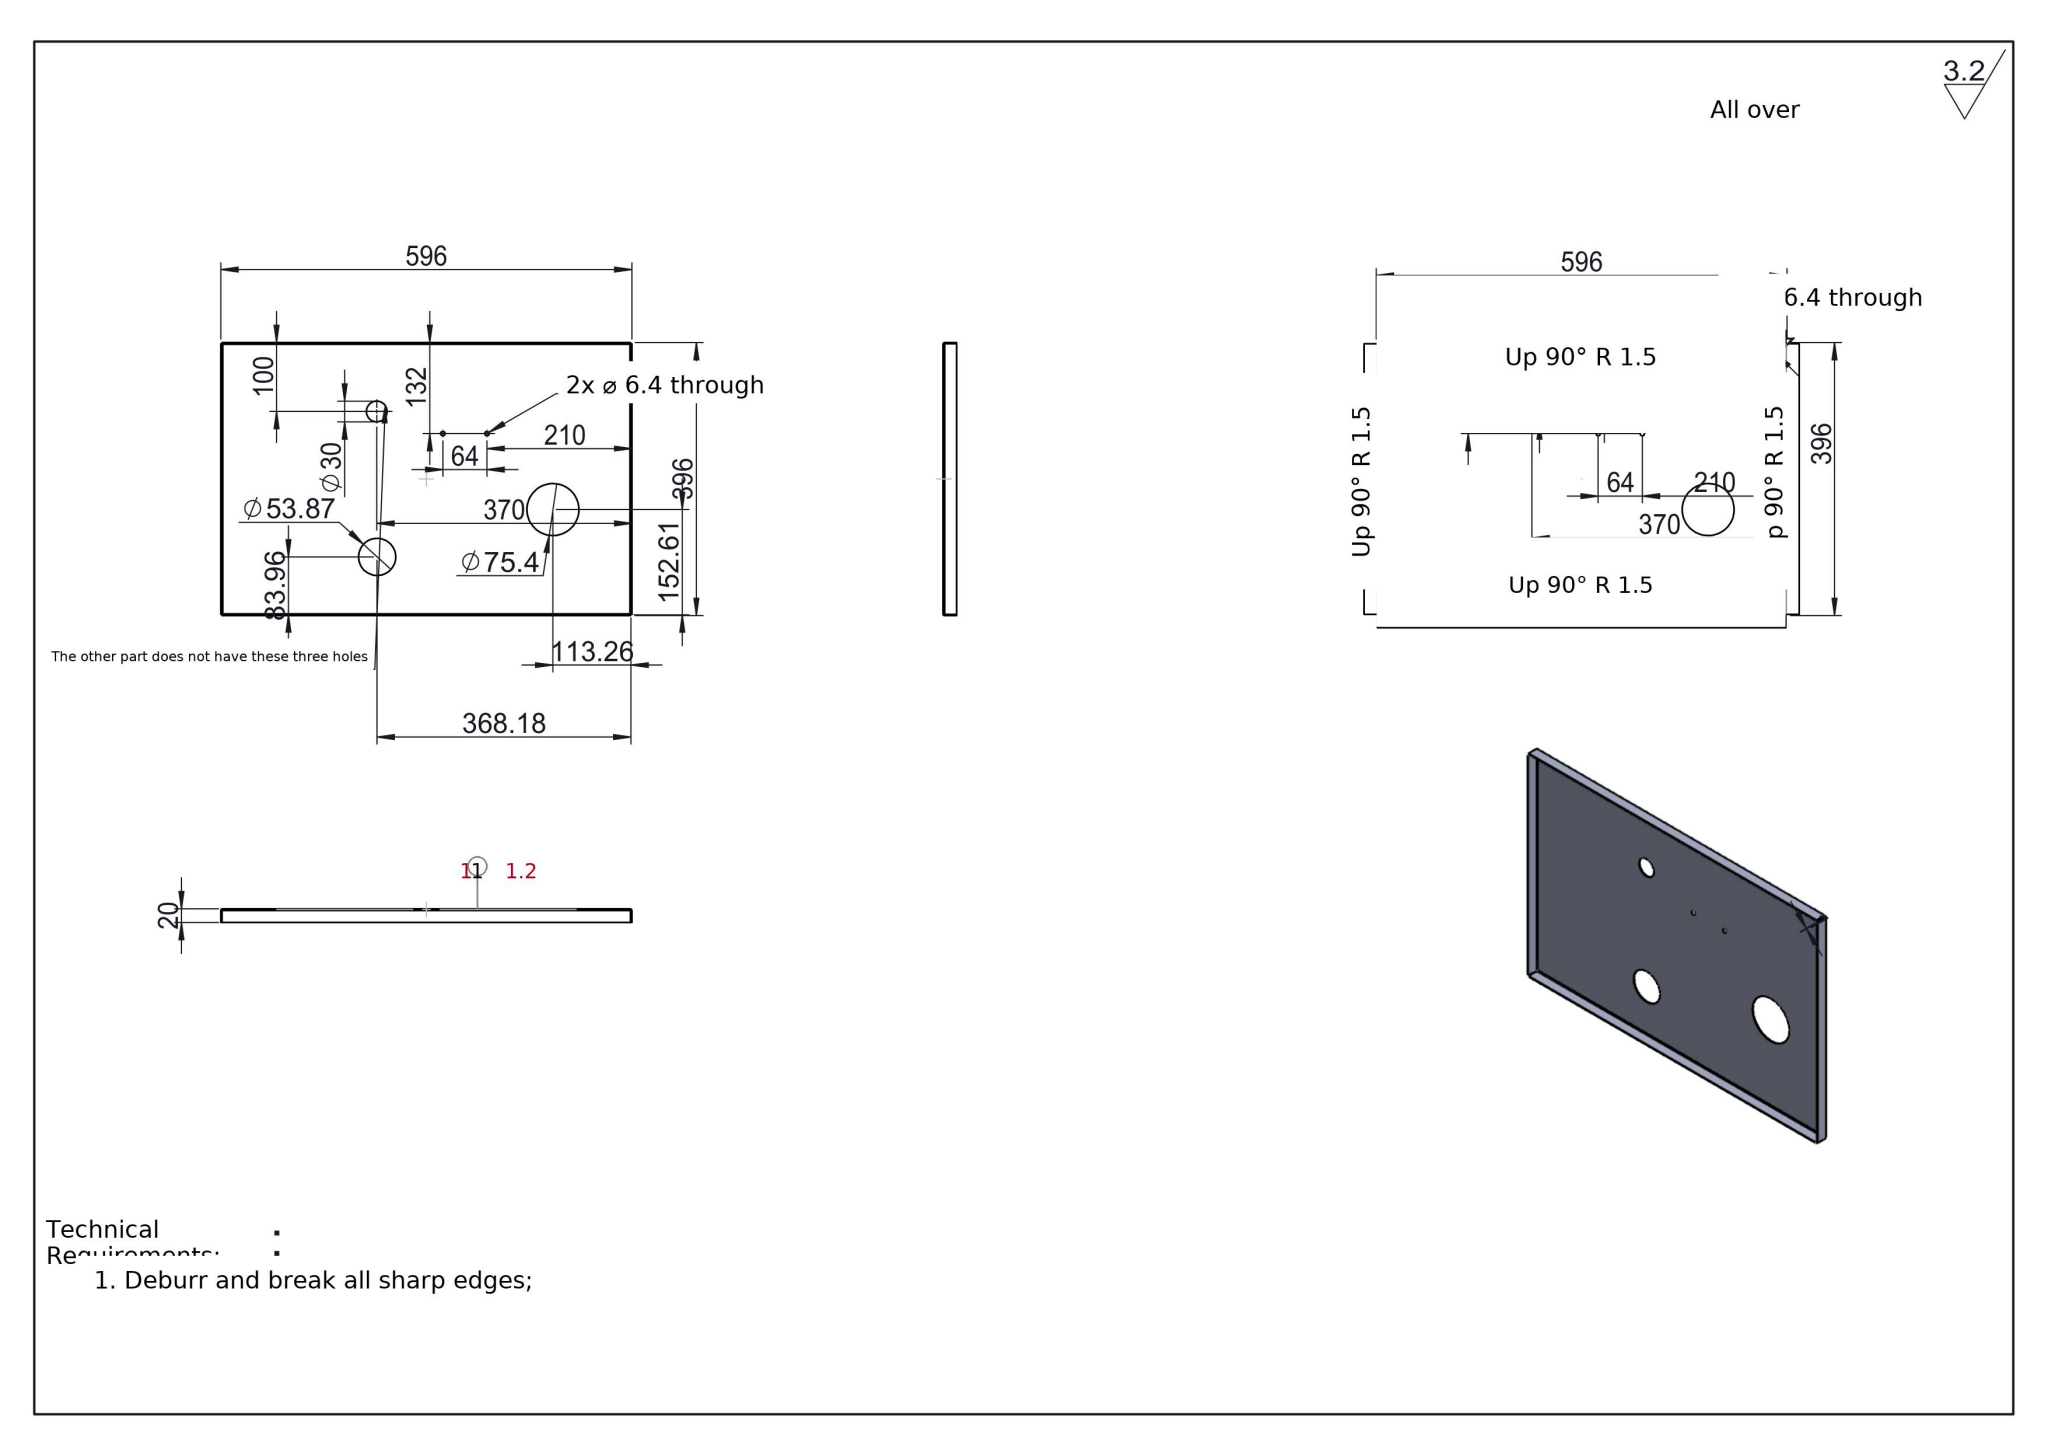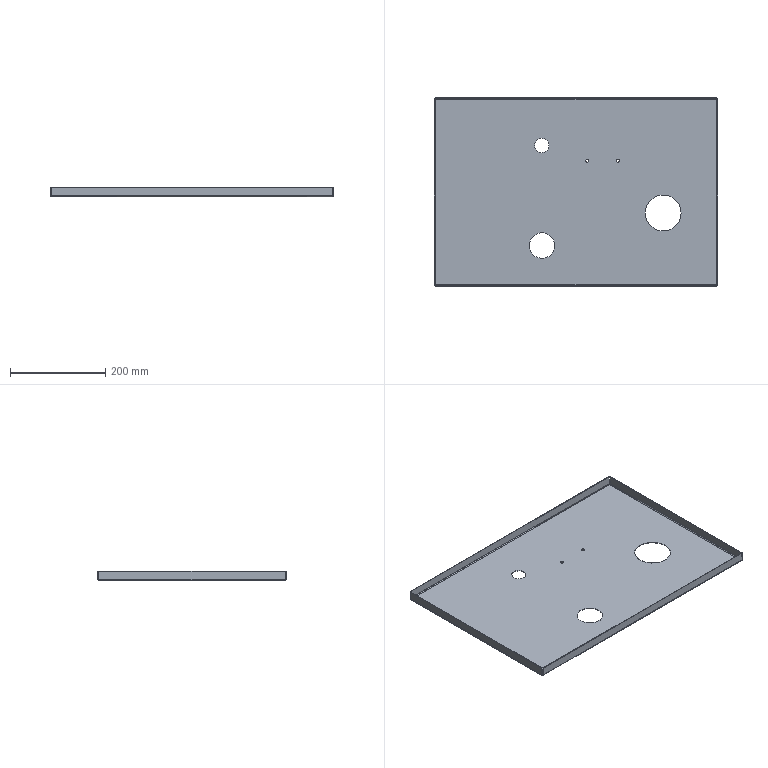Part | SolidWorks | mm | 1 solid | 48 faces | box 596 x 396 x 20 mm | volume 316458 mm3 | plane 22 | cylinder 18 | spline 8 | commonest cylinder face diameters 6.4 x4 5.4 x4 3 x4 75.404 x2 53.87 x2 30 x2